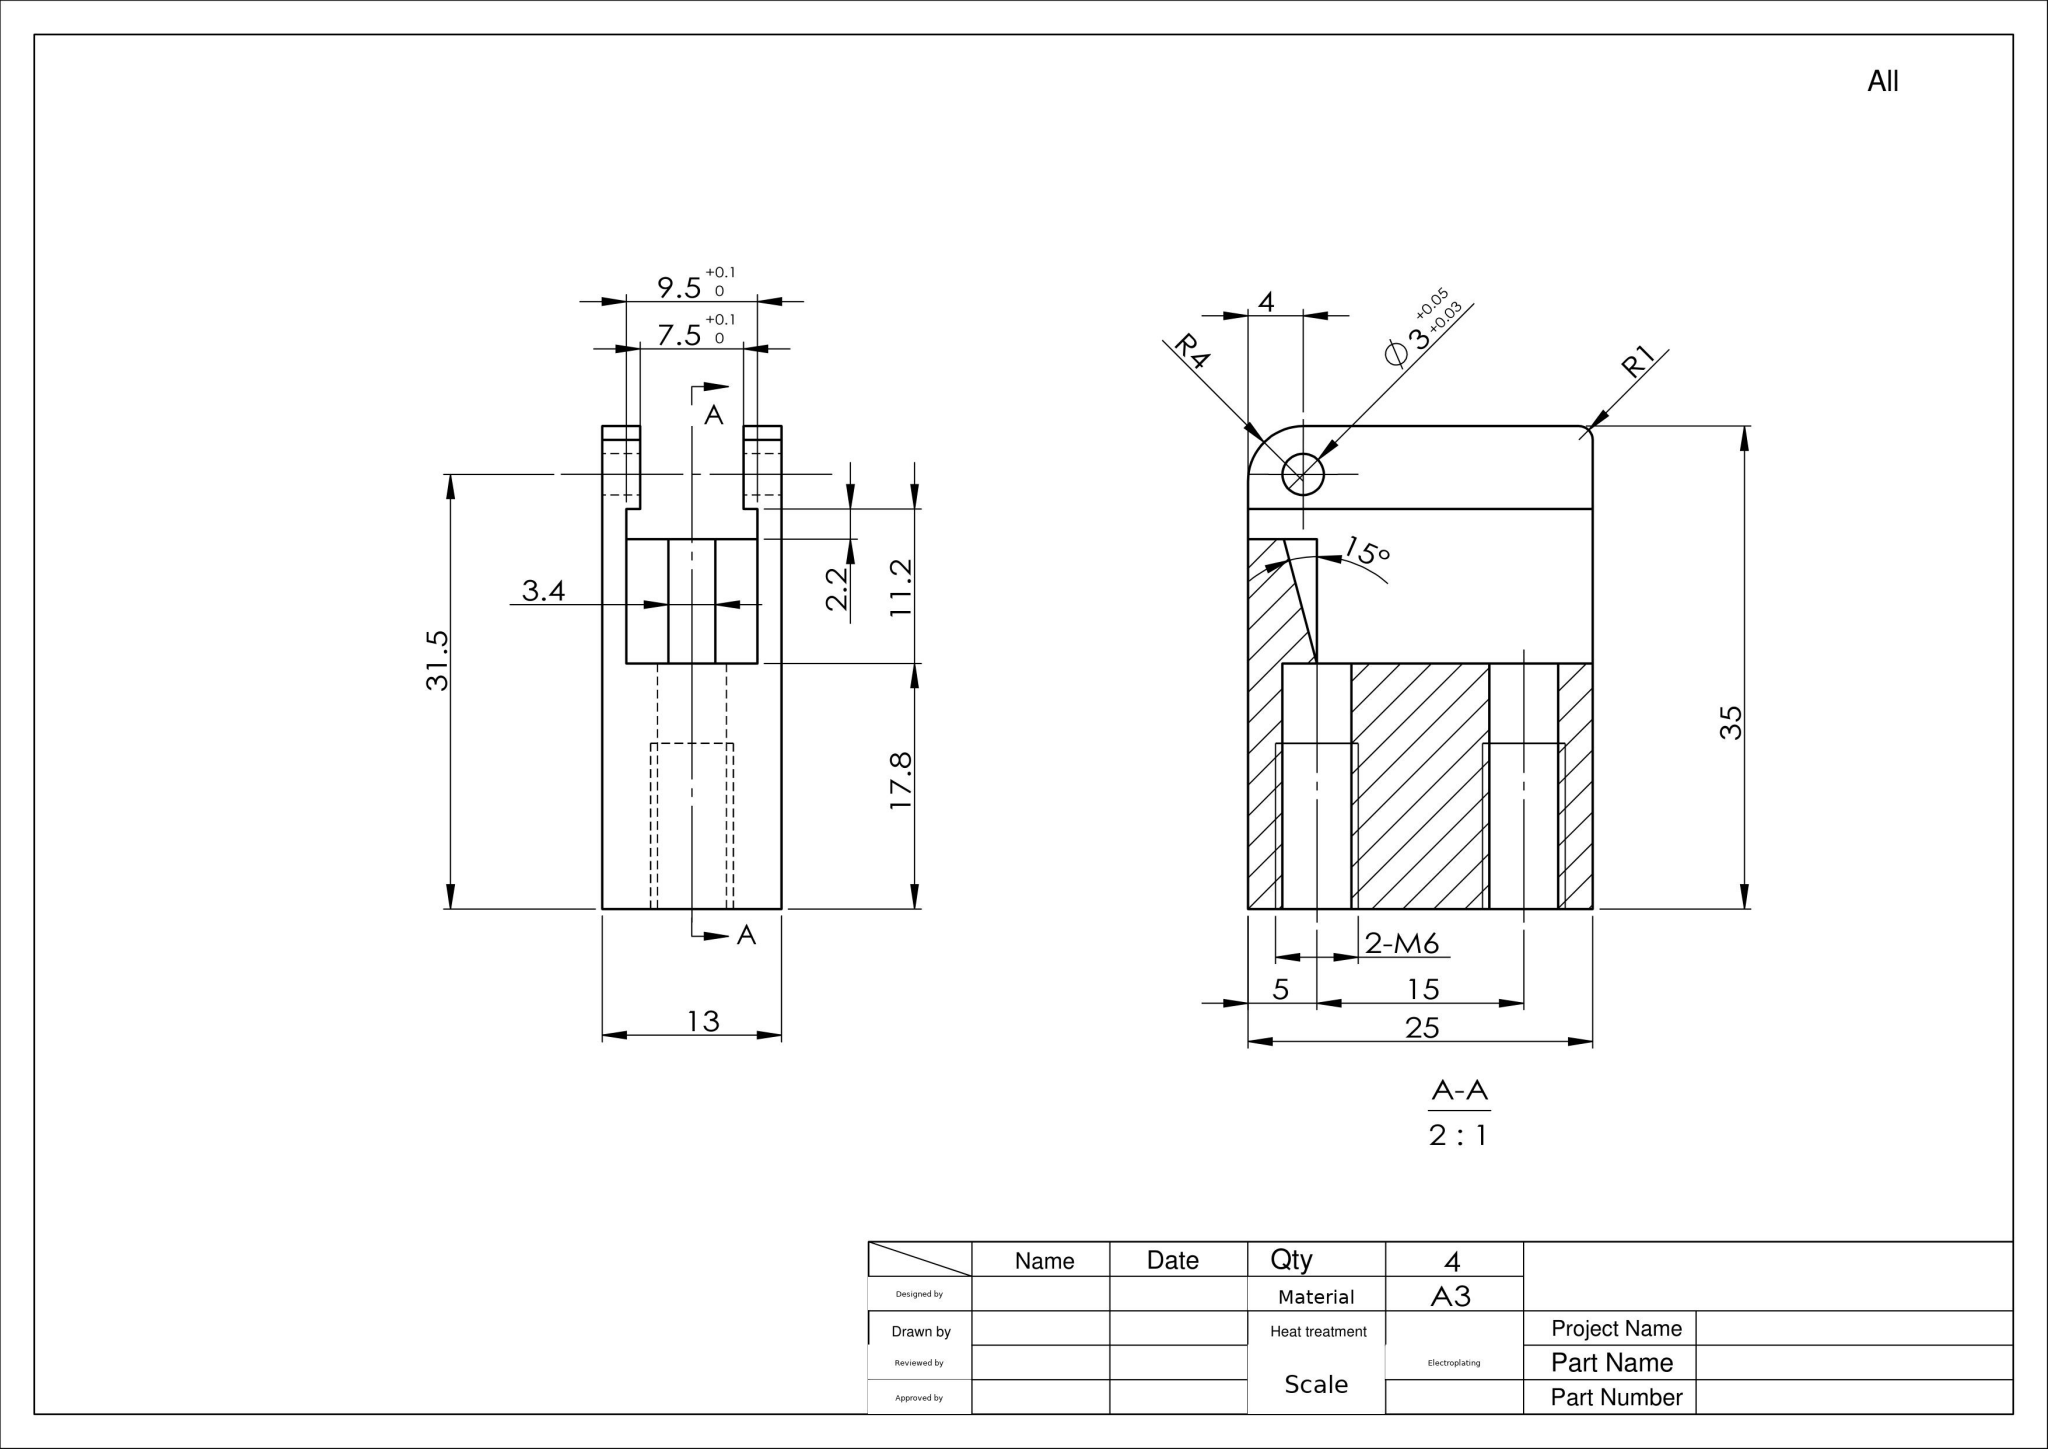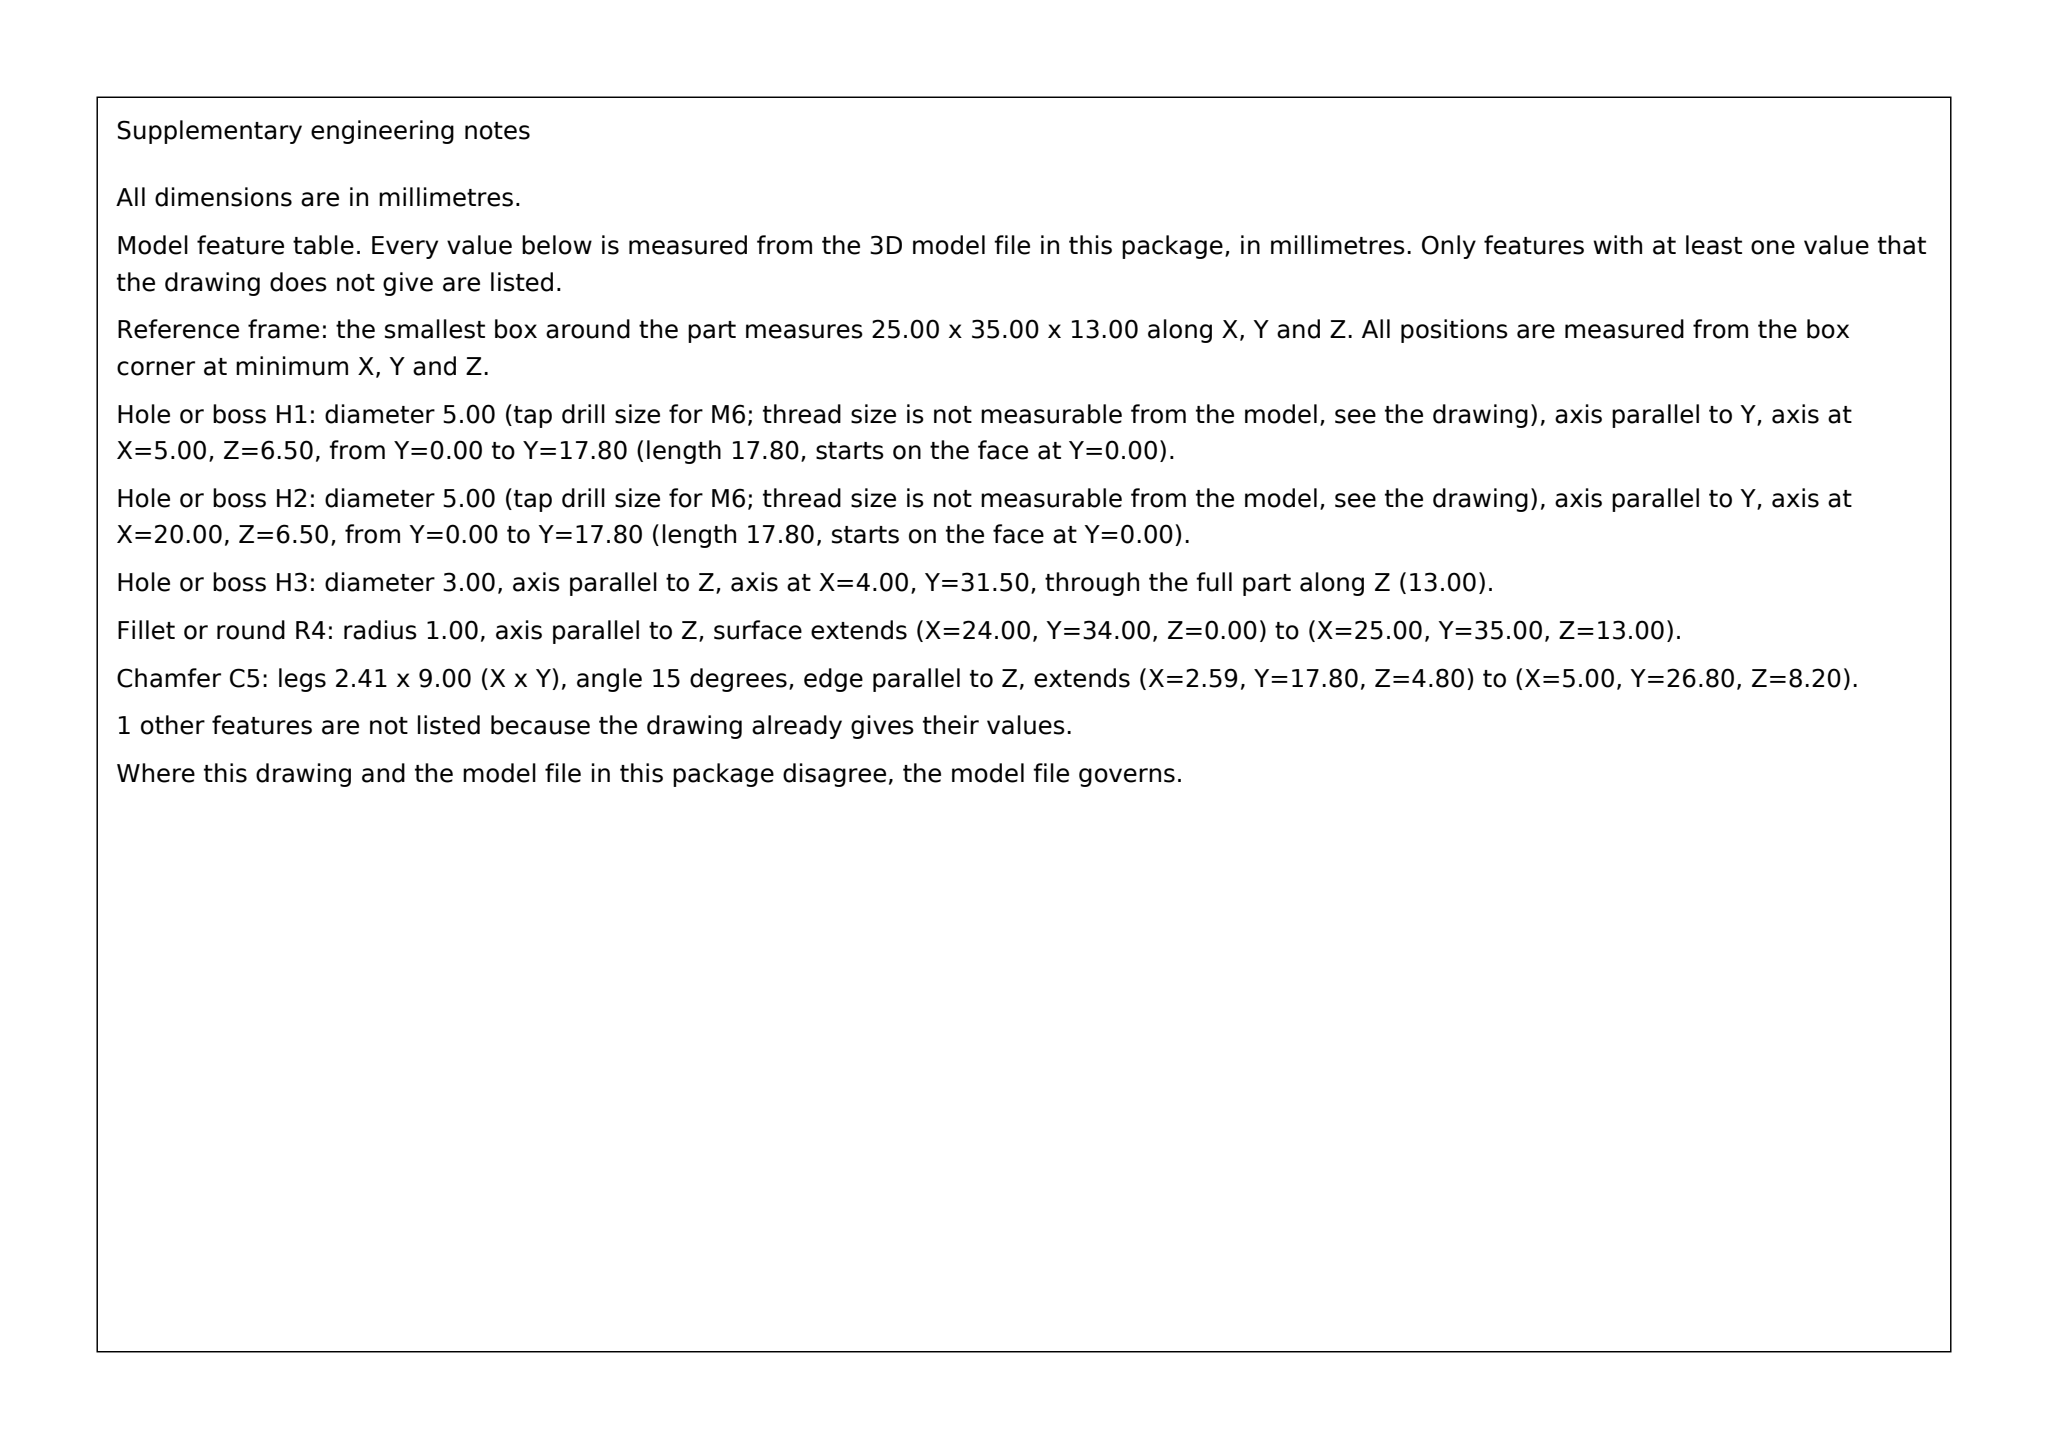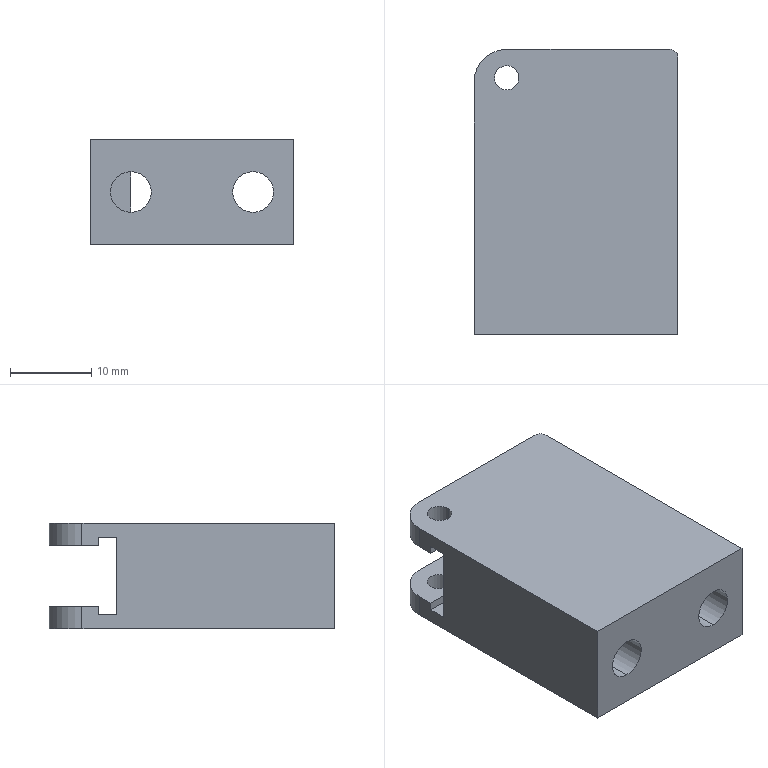Part | SolidWorks | mm | material A3 | 1 solid | 33 faces | box 25 x 35 x 13 mm | volume 7223 mm3 | plane 21 | cylinder 12 | commonest cylinder face diameters 5 x4 3 x4 8 x2 2 x2
build123d program:
from build123d import *

# Parameters (mm, degrees)
SKETCH1_W             = 25
SKETCH1_H             = 35
EXTRUDE1_DEPTH        = 13
CUT_EXTRUDE1_DEPTH    = 20
CUT_EXTRUDE2_DEPTH    = 43.356
CUT_EXTRUDE3_DEPTH    = 1.7
SKETCH6_R             = 1.5
CUT_EXTRUDE4_DEPTH    = 45.933
FILLET1_R             = 4
FILLET2_R             = 1
M6_TAPPED_HOLE1_D     = 5
M6_TAPPED_HOLE1_DEPTH = 17.8


with BuildPart() as part:
    # Sketch1 → Extrude1 (new body)
    with BuildSketch(Plane.XY):
        with Locations((12.5, 17.5)):
            Rectangle(SKETCH1_W, SKETCH1_H)
    extrude(amount=EXTRUDE1_DEPTH)

    # Sketch2 → Cut-Extrude1 (cut)
    with BuildSketch(Plane(origin=(25, 0, 0), x_dir=(0, 0, -1), z_dir=(1, 0, 0))):
        Polygon((-2.75, 29), (-1.75, 29), (-1.75, 17.8), (-11.25, 17.8), (-11.25, 29), (-10.25, 29), (-10.25, 38.13), (-2.75, 38.13), align=None)
    extrude(amount=-CUT_EXTRUDE1_DEPTH, mode=Mode.SUBTRACT)

    # Sketch3 → Cut-Extrude2 (cut, through all)
    with BuildSketch(Plane(origin=(5, 0, 0), x_dir=(0, 0, -1), z_dir=(1, 0, 0))):
        Polygon((-10.25, 35), (-2.75, 35), (-2.75, 29), (-1.75, 29), (-1.75, 26.8), (-11.25, 26.8), (-11.25, 29), (-10.25, 29), align=None)
    extrude(amount=-CUT_EXTRUDE2_DEPTH, mode=Mode.SUBTRACT)

    # Sketch5 → Cut-Extrude3 (cut, symmetric)
    with BuildSketch(Plane(origin=(0, 0, 6.5), x_dir=(-1, 0, 0), z_dir=(0, 0, -1))):
        Polygon((-5, 17.8), (-2.588, 26.8), (-5, 26.8), align=None)
    extrude(amount=CUT_EXTRUDE3_DEPTH, both=True, mode=Mode.SUBTRACT)

    # Sketch6 → Cut-Extrude4 (cut, through all)
    with BuildSketch(Plane(origin=(0, 0, 0), x_dir=(-1, 0, 0), z_dir=(0, 0, -1))):
        with Locations((-4, 31.5)):
            Circle(SKETCH6_R)
    extrude(amount=-CUT_EXTRUDE4_DEPTH, mode=Mode.SUBTRACT)

    # Fillet1
    fillet1_edges = [part.edges().sort_by_distance(p)[0] for p in [
        (0, 35, 1.375),
        (0, 35, 11.625),
    ]]
    fillet(fillet1_edges, radius=FILLET1_R)

    # Fillet2
    fillet2_edges = [part.edges().sort_by_distance(p)[0] for p in [
        (25, 35, 1.375),
        (25, 35, 11.625),
    ]]
    fillet(fillet2_edges, radius=FILLET2_R)

    # M6 Tapped Hole1
    with Locations(Plane(origin=(5, 0, 6.5), x_dir=(0, 0, -1), z_dir=(0, -1, 0))):
        with Locations((0, 0), (0, 15)):
            Hole(M6_TAPPED_HOLE1_D / 2, depth=M6_TAPPED_HOLE1_DEPTH)


solid = part.part